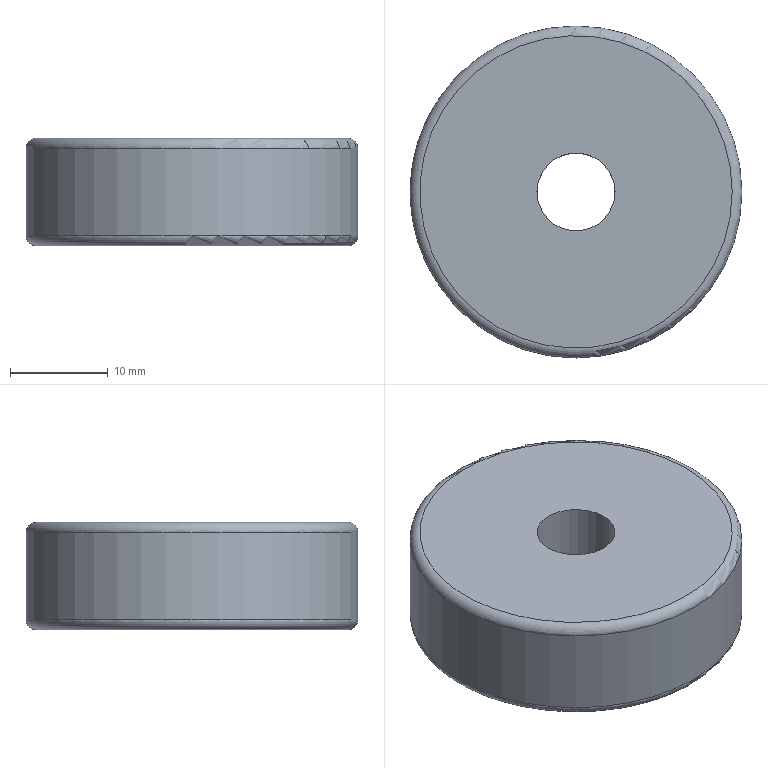Component | NX | BEARING_8_34_2 | 1 solid | 6 faces | box 34 x 34 x 11 mm | volume 9389 mm3 | cylinder 2 | plane 2 | torus 2 | commonest cylinder face diameters 34 x1 8 x1
STEP:
#1=CARTESIAN_POINT('',(0.,0.,0.));
#2=DIRECTION('',(0.,0.,1.));
#3=DIRECTION('',(1.,0.,0.));
#4=AXIS2_PLACEMENT_3D('',#1,#2,#3);
#5=CARTESIAN_POINT('',(642.689,-150.302,-1017.));
#6=VERTEX_POINT('',#5);
#7=CARTESIAN_POINT('',(625.689,-150.302,-1017.));
#8=DIRECTION('',(0.,0.,1.));
#9=DIRECTION('',(1.,0.,0.));
#10=AXIS2_PLACEMENT_3D('',#7,#8,#9);
#11=CIRCLE('',#10,17.);
#12=CARTESIAN_POINT('',(625.689,-150.302,-1007.));
#13=DIRECTION('',(0.,0.,-1.));
#14=DIRECTION('',(-1.,0.,0.));
#15=AXIS2_PLACEMENT_3D('',#12,#13,#14);
#16=CYLINDRICAL_SURFACE('',#15,17.);
#17=CARTESIAN_POINT('',(9.425,10.));
#18=DIRECTION('',(-1.,0.));
#19=VECTOR('',#18,1.);
#20=LINE('',#17,#19);
#21=(GEOMETRIC_REPRESENTATION_CONTEXT(2)PARAMETRIC_REPRESENTATION_CONTEXT()REPRESENTATION_CONTEXT('',''));
#22=DEFINITIONAL_REPRESENTATION('',(#20),#21);
#23=PCURVE('',#16,#22);
#24=CARTESIAN_POINT('',(625.689,-150.302,-1017.));
#25=DIRECTION('',(0.,0.,1.));
#26=DIRECTION('',(1.,0.,0.));
#27=AXIS2_PLACEMENT_3D('',#24,#25,#26);
#28=TOROIDAL_SURFACE('',#27,16.,1.);
#29=CARTESIAN_POINT('',(0.,6.283));
#30=DIRECTION('',(1.,0.));
#31=VECTOR('',#30,1.);
#32=LINE('',#29,#31);
#33=(GEOMETRIC_REPRESENTATION_CONTEXT(2)PARAMETRIC_REPRESENTATION_CONTEXT()REPRESENTATION_CONTEXT('',''));
#34=DEFINITIONAL_REPRESENTATION('',(#32),#33);
#35=PCURVE('',#28,#34);
#36=SURFACE_CURVE('',#11,(#23,#35),.PCURVE_S1.);
#37=EDGE_CURVE('',#6,#6,#36,.T.);
#38=ORIENTED_EDGE('',*,*,#37,.T.);
#39=CARTESIAN_POINT('',(642.689,-150.302,-1008.));
#40=VERTEX_POINT('',#39);
#41=CARTESIAN_POINT('',(642.689,-150.302,-1008.));
#42=CARTESIAN_POINT('',(642.689,-150.302,-1017.));
#43=B_SPLINE_CURVE_WITH_KNOTS('',1,(#41,#42),.UNSPECIFIED.,.F.,.F.,(2,2),(1.,10.),.PIECEWISE_BEZIER_KNOTS.);
#44=CARTESIAN_POINT('',(3.142,0.));
#45=DIRECTION('',(0.,1.));
#46=VECTOR('',#45,1.);
#47=LINE('',#44,#46);
#48=(GEOMETRIC_REPRESENTATION_CONTEXT(2)PARAMETRIC_REPRESENTATION_CONTEXT()REPRESENTATION_CONTEXT('',''));
#49=DEFINITIONAL_REPRESENTATION('',(#47),#48);
#50=PCURVE('',#16,#49);
#51=CARTESIAN_POINT('',(9.425,0.));
#52=DIRECTION('',(0.,1.));
#53=VECTOR('',#52,1.);
#54=LINE('',#51,#53);
#55=(GEOMETRIC_REPRESENTATION_CONTEXT(2)PARAMETRIC_REPRESENTATION_CONTEXT()REPRESENTATION_CONTEXT('',''));
#56=DEFINITIONAL_REPRESENTATION('',(#54),#55);
#57=PCURVE('',#16,#56);
#58=SEAM_CURVE('',#43,(#50,#57),.PCURVE_S1.);
#59=EDGE_CURVE('',#40,#6,#58,.T.);
#60=ORIENTED_EDGE('',*,*,#59,.F.);
#61=CARTESIAN_POINT('',(625.689,-150.302,-1008.));
#62=DIRECTION('',(0.,0.,-1.));
#63=DIRECTION('',(1.,0.,0.));
#64=AXIS2_PLACEMENT_3D('',#61,#62,#63);
#65=CIRCLE('',#64,17.);
#66=CARTESIAN_POINT('',(3.142,1.));
#67=DIRECTION('',(1.,0.));
#68=VECTOR('',#67,1.);
#69=LINE('',#66,#68);
#70=(GEOMETRIC_REPRESENTATION_CONTEXT(2)PARAMETRIC_REPRESENTATION_CONTEXT()REPRESENTATION_CONTEXT('',''));
#71=DEFINITIONAL_REPRESENTATION('',(#69),#70);
#72=PCURVE('',#16,#71);
#73=CARTESIAN_POINT('',(625.689,-150.302,-1008.));
#74=DIRECTION('',(0.,0.,1.));
#75=DIRECTION('',(1.,0.,0.));
#76=AXIS2_PLACEMENT_3D('',#73,#74,#75);
#77=TOROIDAL_SURFACE('',#76,16.,1.);
#78=CARTESIAN_POINT('',(6.283,6.283));
#79=DIRECTION('',(-1.,0.));
#80=VECTOR('',#79,1.);
#81=LINE('',#78,#80);
#82=(GEOMETRIC_REPRESENTATION_CONTEXT(2)PARAMETRIC_REPRESENTATION_CONTEXT()REPRESENTATION_CONTEXT('',''));
#83=DEFINITIONAL_REPRESENTATION('',(#81),#82);
#84=PCURVE('',#77,#83);
#85=SURFACE_CURVE('',#65,(#72,#84),.PCURVE_S1.);
#86=EDGE_CURVE('',#40,#40,#85,.T.);
#87=ORIENTED_EDGE('',*,*,#86,.T.);
#88=ORIENTED_EDGE('',*,*,#59,.T.);
#89=EDGE_LOOP('',(#38,#60,#87,#88));
#90=FACE_BOUND('',#89,.T.);
#91=ADVANCED_FACE('',(#90),#16,.T.);
#92=CARTESIAN_POINT('',(629.689,-150.302,-1007.));
#93=VERTEX_POINT('',#92);
#94=CARTESIAN_POINT('',(625.689,-150.302,-1007.));
#95=DIRECTION('',(0.,0.,1.));
#96=DIRECTION('',(1.,0.,0.));
#97=AXIS2_PLACEMENT_3D('',#94,#95,#96);
#98=CIRCLE('',#97,4.);
#99=CARTESIAN_POINT('',(625.689,-150.302,-1007.));
#100=DIRECTION('',(0.,0.,-1.));
#101=DIRECTION('',(-1.,0.,0.));
#102=AXIS2_PLACEMENT_3D('',#99,#100,#101);
#103=CYLINDRICAL_SURFACE('',#102,4.);
#104=CARTESIAN_POINT('',(9.425,0.));
#105=DIRECTION('',(-1.,0.));
#106=VECTOR('',#105,1.);
#107=LINE('',#104,#106);
#108=(GEOMETRIC_REPRESENTATION_CONTEXT(2)PARAMETRIC_REPRESENTATION_CONTEXT()REPRESENTATION_CONTEXT('',''));
#109=DEFINITIONAL_REPRESENTATION('',(#107),#108);
#110=PCURVE('',#103,#109);
#111=CARTESIAN_POINT('',(625.689,-150.302,-1007.));
#112=DIRECTION('',(0.,0.,1.));
#113=DIRECTION('',(1.,0.,0.));
#114=AXIS2_PLACEMENT_3D('',#111,#112,#113);
#115=PLANE('',#114);
#116=CARTESIAN_POINT('',(0.,0.));
#117=DIRECTION('',(1.,0.));
#118=AXIS2_PLACEMENT_2D('',#116,#117);
#119=CIRCLE('',#118,4.);
#120=(GEOMETRIC_REPRESENTATION_CONTEXT(2)PARAMETRIC_REPRESENTATION_CONTEXT()REPRESENTATION_CONTEXT('',''));
#121=DEFINITIONAL_REPRESENTATION('',(#119),#120);
#122=PCURVE('',#115,#121);
#123=SURFACE_CURVE('',#98,(#110,#122),.PCURVE_S1.);
#124=EDGE_CURVE('',#93,#93,#123,.T.);
#125=ORIENTED_EDGE('',*,*,#124,.F.);
#126=CARTESIAN_POINT('',(629.689,-150.302,-1018.));
#127=VERTEX_POINT('',#126);
#128=CARTESIAN_POINT('',(629.689,-150.302,-1007.));
#129=CARTESIAN_POINT('',(629.689,-150.302,-1018.));
#130=B_SPLINE_CURVE_WITH_KNOTS('',1,(#128,#129),.UNSPECIFIED.,.F.,.F.,(2,2),(0.,11.),.PIECEWISE_BEZIER_KNOTS.);
#131=CARTESIAN_POINT('',(9.425,0.));
#132=DIRECTION('',(0.,1.));
#133=VECTOR('',#132,1.);
#134=LINE('',#131,#133);
#135=(GEOMETRIC_REPRESENTATION_CONTEXT(2)PARAMETRIC_REPRESENTATION_CONTEXT()REPRESENTATION_CONTEXT('',''));
#136=DEFINITIONAL_REPRESENTATION('',(#134),#135);
#137=PCURVE('',#103,#136);
#138=CARTESIAN_POINT('',(3.142,0.));
#139=DIRECTION('',(0.,1.));
#140=VECTOR('',#139,1.);
#141=LINE('',#138,#140);
#142=(GEOMETRIC_REPRESENTATION_CONTEXT(2)PARAMETRIC_REPRESENTATION_CONTEXT()REPRESENTATION_CONTEXT('',''));
#143=DEFINITIONAL_REPRESENTATION('',(#141),#142);
#144=PCURVE('',#103,#143);
#145=SEAM_CURVE('',#130,(#137,#144),.PCURVE_S1.);
#146=EDGE_CURVE('',#93,#127,#145,.T.);
#147=ORIENTED_EDGE('',*,*,#146,.T.);
#148=CARTESIAN_POINT('',(625.689,-150.302,-1018.));
#149=DIRECTION('',(0.,0.,1.));
#150=DIRECTION('',(1.,0.,0.));
#151=AXIS2_PLACEMENT_3D('',#148,#149,#150);
#152=CIRCLE('',#151,4.);
#153=CARTESIAN_POINT('',(9.425,11.));
#154=DIRECTION('',(-1.,0.));
#155=VECTOR('',#154,1.);
#156=LINE('',#153,#155);
#157=(GEOMETRIC_REPRESENTATION_CONTEXT(2)PARAMETRIC_REPRESENTATION_CONTEXT()REPRESENTATION_CONTEXT('',''));
#158=DEFINITIONAL_REPRESENTATION('',(#156),#157);
#159=PCURVE('',#103,#158);
#160=CARTESIAN_POINT('',(625.689,-150.302,-1018.));
#161=DIRECTION('',(0.,0.,1.));
#162=DIRECTION('',(1.,0.,0.));
#163=AXIS2_PLACEMENT_3D('',#160,#161,#162);
#164=PLANE('',#163);
#165=CARTESIAN_POINT('',(0.,0.));
#166=DIRECTION('',(1.,0.));
#167=AXIS2_PLACEMENT_2D('',#165,#166);
#168=CIRCLE('',#167,4.);
#169=(GEOMETRIC_REPRESENTATION_CONTEXT(2)PARAMETRIC_REPRESENTATION_CONTEXT()REPRESENTATION_CONTEXT('',''));
#170=DEFINITIONAL_REPRESENTATION('',(#168),#169);
#171=PCURVE('',#164,#170);
#172=SURFACE_CURVE('',#152,(#159,#171),.PCURVE_S1.);
#173=EDGE_CURVE('',#127,#127,#172,.T.);
#174=ORIENTED_EDGE('',*,*,#173,.T.);
#175=ORIENTED_EDGE('',*,*,#146,.F.);
#176=EDGE_LOOP('',(#125,#147,#174,#175));
#177=FACE_BOUND('',#176,.F.);
#178=ADVANCED_FACE('',(#177),#103,.F.);
#179=CARTESIAN_POINT('',(641.689,-150.302,-1007.));
#180=VERTEX_POINT('',#179);
#181=CARTESIAN_POINT('',(625.689,-150.302,-1007.));
#182=DIRECTION('',(0.,0.,1.));
#183=DIRECTION('',(1.,0.,0.));
#184=AXIS2_PLACEMENT_3D('',#181,#182,#183);
#185=CIRCLE('',#184,16.);
#186=CARTESIAN_POINT('',(0.,0.));
#187=DIRECTION('',(1.,0.));
#188=AXIS2_PLACEMENT_2D('',#186,#187);
#189=CIRCLE('',#188,16.);
#190=(GEOMETRIC_REPRESENTATION_CONTEXT(2)PARAMETRIC_REPRESENTATION_CONTEXT()REPRESENTATION_CONTEXT('',''));
#191=DEFINITIONAL_REPRESENTATION('',(#189),#190);
#192=PCURVE('',#115,#191);
#193=CARTESIAN_POINT('',(0.,7.854));
#194=DIRECTION('',(1.,0.));
#195=VECTOR('',#194,1.);
#196=LINE('',#193,#195);
#197=(GEOMETRIC_REPRESENTATION_CONTEXT(2)PARAMETRIC_REPRESENTATION_CONTEXT()REPRESENTATION_CONTEXT('',''));
#198=DEFINITIONAL_REPRESENTATION('',(#196),#197);
#199=PCURVE('',#77,#198);
#200=SURFACE_CURVE('',#185,(#192,#199),.PCURVE_S1.);
#201=EDGE_CURVE('',#180,#180,#200,.T.);
#202=ORIENTED_EDGE('',*,*,#201,.T.);
#203=EDGE_LOOP('',(#202));
#204=FACE_BOUND('',#203,.T.);
#205=ORIENTED_EDGE('',*,*,#124,.F.);
#206=EDGE_LOOP('',(#205));
#207=FACE_BOUND('',#206,.T.);
#208=ADVANCED_FACE('',(#204,#207),#115,.T.);
#209=CARTESIAN_POINT('',(641.689,-150.302,-1018.));
#210=VERTEX_POINT('',#209);
#211=CARTESIAN_POINT('',(625.689,-150.302,-1018.));
#212=DIRECTION('',(0.,0.,-1.));
#213=DIRECTION('',(1.,0.,0.));
#214=AXIS2_PLACEMENT_3D('',#211,#212,#213);
#215=CIRCLE('',#214,16.);
#216=CARTESIAN_POINT('',(16.,0.));
#217=CARTESIAN_POINT('',(16.,-27.713));
#218=CARTESIAN_POINT('',(-8.,-13.856));
#219=CARTESIAN_POINT('',(-32.,-0.));
#220=CARTESIAN_POINT('',(-8.,13.856));
#221=CARTESIAN_POINT('',(16.,27.713));
#222=CARTESIAN_POINT('',(16.,0.));
#223=(BOUNDED_CURVE()B_SPLINE_CURVE(2,(#216,#217,#218,#219,#220,#221,#222),.UNSPECIFIED.,.T.,.F.)B_SPLINE_CURVE_WITH_KNOTS((1,2,2,2,2,1),(-2.094,0.,2.094,4.189,6.283,8.378),.UNSPECIFIED.)CURVE()GEOMETRIC_REPRESENTATION_ITEM()RATIONAL_B_SPLINE_CURVE((1.,0.5,1.,0.5,1.,0.5,1.))REPRESENTATION_ITEM(''));
#224=(GEOMETRIC_REPRESENTATION_CONTEXT(2)PARAMETRIC_REPRESENTATION_CONTEXT()REPRESENTATION_CONTEXT('',''));
#225=DEFINITIONAL_REPRESENTATION('',(#223),#224);
#226=PCURVE('',#164,#225);
#227=CARTESIAN_POINT('',(6.283,4.712));
#228=DIRECTION('',(-1.,0.));
#229=VECTOR('',#228,1.);
#230=LINE('',#227,#229);
#231=(GEOMETRIC_REPRESENTATION_CONTEXT(2)PARAMETRIC_REPRESENTATION_CONTEXT()REPRESENTATION_CONTEXT('',''));
#232=DEFINITIONAL_REPRESENTATION('',(#230),#231);
#233=PCURVE('',#28,#232);
#234=SURFACE_CURVE('',#215,(#226,#233),.PCURVE_S1.);
#235=EDGE_CURVE('',#210,#210,#234,.T.);
#236=ORIENTED_EDGE('',*,*,#235,.T.);
#237=EDGE_LOOP('',(#236));
#238=FACE_BOUND('',#237,.T.);
#239=ORIENTED_EDGE('',*,*,#173,.T.);
#240=EDGE_LOOP('',(#239));
#241=FACE_BOUND('',#240,.T.);
#242=ADVANCED_FACE('',(#238,#241),#164,.F.);
#243=ORIENTED_EDGE('',*,*,#235,.F.);
#244=CARTESIAN_POINT('',(641.689,-150.302,-1018.));
#245=CARTESIAN_POINT('',(641.956,-150.302,-1018.));
#246=CARTESIAN_POINT('',(642.217,-150.302,-1017.915));
#247=CARTESIAN_POINT('',(642.441,-150.302,-1017.752));
#248=CARTESIAN_POINT('',(642.604,-150.302,-1017.528));
#249=CARTESIAN_POINT('',(642.689,-150.302,-1017.267));
#250=CARTESIAN_POINT('',(642.689,-150.302,-1017.));
#251=(BOUNDED_CURVE()B_SPLINE_CURVE(6,(#244,#245,#246,#247,#248,#249,#250),.UNSPECIFIED.,.F.,.F.)B_SPLINE_CURVE_WITH_KNOTS((7,7),(4.712,6.283),.PIECEWISE_BEZIER_KNOTS.)CURVE()GEOMETRIC_REPRESENTATION_ITEM()RATIONAL_B_SPLINE_CURVE((1.031,1.01,0.9979,0.994,0.9979,1.01,1.031))REPRESENTATION_ITEM(''));
#252=CARTESIAN_POINT('',(6.283,0.));
#253=DIRECTION('',(0.,1.));
#254=VECTOR('',#253,1.);
#255=LINE('',#252,#254);
#256=(GEOMETRIC_REPRESENTATION_CONTEXT(2)PARAMETRIC_REPRESENTATION_CONTEXT()REPRESENTATION_CONTEXT('',''));
#257=DEFINITIONAL_REPRESENTATION('',(#255),#256);
#258=PCURVE('',#28,#257);
#259=CARTESIAN_POINT('',(0.,0.));
#260=DIRECTION('',(0.,1.));
#261=VECTOR('',#260,1.);
#262=LINE('',#259,#261);
#263=(GEOMETRIC_REPRESENTATION_CONTEXT(2)PARAMETRIC_REPRESENTATION_CONTEXT()REPRESENTATION_CONTEXT('',''));
#264=DEFINITIONAL_REPRESENTATION('',(#262),#263);
#265=PCURVE('',#28,#264);
#266=SEAM_CURVE('',#251,(#258,#265),.PCURVE_S1.);
#267=EDGE_CURVE('',#210,#6,#266,.T.);
#268=ORIENTED_EDGE('',*,*,#267,.T.);
#269=ORIENTED_EDGE('',*,*,#37,.F.);
#270=ORIENTED_EDGE('',*,*,#267,.F.);
#271=EDGE_LOOP('',(#243,#268,#269,#270));
#272=FACE_BOUND('',#271,.T.);
#273=ADVANCED_FACE('',(#272),#28,.T.);
#274=ORIENTED_EDGE('',*,*,#86,.F.);
#275=CARTESIAN_POINT('',(642.689,-150.302,-1008.));
#276=CARTESIAN_POINT('',(642.689,-150.302,-1007.733));
#277=CARTESIAN_POINT('',(642.604,-150.302,-1007.472));
#278=CARTESIAN_POINT('',(642.441,-150.302,-1007.248));
#279=CARTESIAN_POINT('',(642.217,-150.302,-1007.085));
#280=CARTESIAN_POINT('',(641.956,-150.302,-1007.));
#281=CARTESIAN_POINT('',(641.689,-150.302,-1007.));
#282=(BOUNDED_CURVE()B_SPLINE_CURVE(6,(#275,#276,#277,#278,#279,#280,#281),.UNSPECIFIED.,.F.,.F.)B_SPLINE_CURVE_WITH_KNOTS((7,7),(0.,1.571),.PIECEWISE_BEZIER_KNOTS.)CURVE()GEOMETRIC_REPRESENTATION_ITEM()RATIONAL_B_SPLINE_CURVE((1.031,1.01,0.9979,0.994,0.9979,1.01,1.031))REPRESENTATION_ITEM(''));
#283=CARTESIAN_POINT('',(6.283,6.283));
#284=DIRECTION('',(0.,1.));
#285=VECTOR('',#284,1.);
#286=LINE('',#283,#285);
#287=(GEOMETRIC_REPRESENTATION_CONTEXT(2)PARAMETRIC_REPRESENTATION_CONTEXT()REPRESENTATION_CONTEXT('',''));
#288=DEFINITIONAL_REPRESENTATION('',(#286),#287);
#289=PCURVE('',#77,#288);
#290=CARTESIAN_POINT('',(0.,6.283));
#291=DIRECTION('',(0.,1.));
#292=VECTOR('',#291,1.);
#293=LINE('',#290,#292);
#294=(GEOMETRIC_REPRESENTATION_CONTEXT(2)PARAMETRIC_REPRESENTATION_CONTEXT()REPRESENTATION_CONTEXT('',''));
#295=DEFINITIONAL_REPRESENTATION('',(#293),#294);
#296=PCURVE('',#77,#295);
#297=SEAM_CURVE('',#282,(#289,#296),.PCURVE_S1.);
#298=EDGE_CURVE('',#40,#180,#297,.T.);
#299=ORIENTED_EDGE('',*,*,#298,.T.);
#300=ORIENTED_EDGE('',*,*,#201,.F.);
#301=ORIENTED_EDGE('',*,*,#298,.F.);
#302=EDGE_LOOP('',(#274,#299,#300,#301));
#303=FACE_BOUND('',#302,.T.);
#304=ADVANCED_FACE('',(#303),#77,.T.);
#305=CLOSED_SHELL('',(#91,#178,#208,#242,#273,#304));
#306=MANIFOLD_SOLID_BREP('',#305);
#307=(LENGTH_UNIT()NAMED_UNIT(*)SI_UNIT(.MILLI.,.METRE.));
#308=UNCERTAINTY_MEASURE_WITH_UNIT(LENGTH_MEASURE(0.00001),#307,'','');
#309=(NAMED_UNIT(*)PLANE_ANGLE_UNIT()SI_UNIT($,.RADIAN.));
#310=(NAMED_UNIT(*)SI_UNIT($,.STERADIAN.)SOLID_ANGLE_UNIT());
#311=(GEOMETRIC_REPRESENTATION_CONTEXT(3)GLOBAL_UNCERTAINTY_ASSIGNED_CONTEXT((#308))GLOBAL_UNIT_ASSIGNED_CONTEXT((#307,#309,#310))REPRESENTATION_CONTEXT('',''));
#312=ADVANCED_BREP_SHAPE_REPRESENTATION('',(#4,#306),#311);